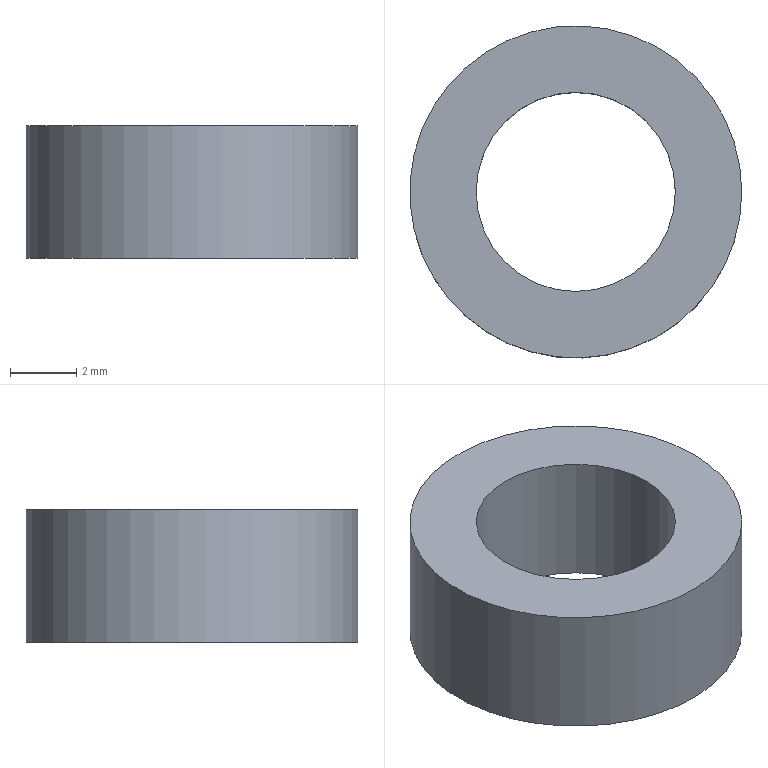Component | NX | BOTTOM_PLATE_WASHER | 1 solid | 4 faces | box 10 x 10 x 4 mm | volume 201 mm3 | cylinder 2 | plane 2 | commonest cylinder face diameters 10 x1 6 x1
STEP:
#1=CARTESIAN_POINT('',(0.,0.,0.));
#2=DIRECTION('',(0.,0.,1.));
#3=DIRECTION('',(1.,0.,0.));
#4=AXIS2_PLACEMENT_3D('',#1,#2,#3);
#5=CARTESIAN_POINT('',(5.,-10.,117.5));
#6=VERTEX_POINT('',#5);
#7=CARTESIAN_POINT('',(-0.,-10.,117.5));
#8=DIRECTION('',(0.,0.,1.));
#9=DIRECTION('',(1.,0.,0.));
#10=AXIS2_PLACEMENT_3D('',#7,#8,#9);
#11=CIRCLE('',#10,5.);
#12=CARTESIAN_POINT('',(-0.,-10.,117.5));
#13=DIRECTION('',(0.,0.,1.));
#14=DIRECTION('',(-1.,0.,0.));
#15=AXIS2_PLACEMENT_3D('',#12,#13,#14);
#16=CYLINDRICAL_SURFACE('',#15,5.);
#17=CARTESIAN_POINT('',(3.142,0.));
#18=DIRECTION('',(1.,0.));
#19=VECTOR('',#18,1.);
#20=LINE('',#17,#19);
#21=(GEOMETRIC_REPRESENTATION_CONTEXT(2)PARAMETRIC_REPRESENTATION_CONTEXT()REPRESENTATION_CONTEXT('',''));
#22=DEFINITIONAL_REPRESENTATION('',(#20),#21);
#23=PCURVE('',#16,#22);
#24=CARTESIAN_POINT('',(-0.,-10.,117.5));
#25=DIRECTION('',(0.,0.,1.));
#26=DIRECTION('',(-1.,0.,0.));
#27=AXIS2_PLACEMENT_3D('',#24,#25,#26);
#28=PLANE('',#27);
#29=CARTESIAN_POINT('',(0.,0.));
#30=DIRECTION('',(-1.,0.));
#31=AXIS2_PLACEMENT_2D('',#29,#30);
#32=CIRCLE('',#31,5.);
#33=(GEOMETRIC_REPRESENTATION_CONTEXT(2)PARAMETRIC_REPRESENTATION_CONTEXT()REPRESENTATION_CONTEXT('',''));
#34=DEFINITIONAL_REPRESENTATION('',(#32),#33);
#35=PCURVE('',#28,#34);
#36=SURFACE_CURVE('',#11,(#23,#35),.PCURVE_S1.);
#37=EDGE_CURVE('',#6,#6,#36,.T.);
#38=ORIENTED_EDGE('',*,*,#37,.T.);
#39=CARTESIAN_POINT('',(5.,-10.,121.5));
#40=VERTEX_POINT('',#39);
#41=CARTESIAN_POINT('',(5.,-10.,117.5));
#42=CARTESIAN_POINT('',(5.,-10.,121.5));
#43=B_SPLINE_CURVE_WITH_KNOTS('',1,(#41,#42),.UNSPECIFIED.,.F.,.F.,(2,2),(0.,4.),.PIECEWISE_BEZIER_KNOTS.);
#44=CARTESIAN_POINT('',(9.425,0.));
#45=DIRECTION('',(0.,1.));
#46=VECTOR('',#45,1.);
#47=LINE('',#44,#46);
#48=(GEOMETRIC_REPRESENTATION_CONTEXT(2)PARAMETRIC_REPRESENTATION_CONTEXT()REPRESENTATION_CONTEXT('',''));
#49=DEFINITIONAL_REPRESENTATION('',(#47),#48);
#50=PCURVE('',#16,#49);
#51=CARTESIAN_POINT('',(3.142,0.));
#52=DIRECTION('',(0.,1.));
#53=VECTOR('',#52,1.);
#54=LINE('',#51,#53);
#55=(GEOMETRIC_REPRESENTATION_CONTEXT(2)PARAMETRIC_REPRESENTATION_CONTEXT()REPRESENTATION_CONTEXT('',''));
#56=DEFINITIONAL_REPRESENTATION('',(#54),#55);
#57=PCURVE('',#16,#56);
#58=SEAM_CURVE('',#43,(#50,#57),.PCURVE_S1.);
#59=EDGE_CURVE('',#6,#40,#58,.T.);
#60=ORIENTED_EDGE('',*,*,#59,.T.);
#61=CARTESIAN_POINT('',(-0.,-10.,121.5));
#62=DIRECTION('',(0.,0.,1.));
#63=DIRECTION('',(1.,0.,0.));
#64=AXIS2_PLACEMENT_3D('',#61,#62,#63);
#65=CIRCLE('',#64,5.);
#66=CARTESIAN_POINT('',(3.142,4.));
#67=DIRECTION('',(1.,0.));
#68=VECTOR('',#67,1.);
#69=LINE('',#66,#68);
#70=(GEOMETRIC_REPRESENTATION_CONTEXT(2)PARAMETRIC_REPRESENTATION_CONTEXT()REPRESENTATION_CONTEXT('',''));
#71=DEFINITIONAL_REPRESENTATION('',(#69),#70);
#72=PCURVE('',#16,#71);
#73=CARTESIAN_POINT('',(-0.,-10.,121.5));
#74=DIRECTION('',(0.,0.,1.));
#75=DIRECTION('',(-1.,0.,0.));
#76=AXIS2_PLACEMENT_3D('',#73,#74,#75);
#77=PLANE('',#76);
#78=CARTESIAN_POINT('',(0.,0.));
#79=DIRECTION('',(-1.,0.));
#80=AXIS2_PLACEMENT_2D('',#78,#79);
#81=CIRCLE('',#80,5.);
#82=(GEOMETRIC_REPRESENTATION_CONTEXT(2)PARAMETRIC_REPRESENTATION_CONTEXT()REPRESENTATION_CONTEXT('',''));
#83=DEFINITIONAL_REPRESENTATION('',(#81),#82);
#84=PCURVE('',#77,#83);
#85=SURFACE_CURVE('',#65,(#72,#84),.PCURVE_S1.);
#86=EDGE_CURVE('',#40,#40,#85,.T.);
#87=ORIENTED_EDGE('',*,*,#86,.F.);
#88=ORIENTED_EDGE('',*,*,#59,.F.);
#89=EDGE_LOOP('',(#38,#60,#87,#88));
#90=FACE_BOUND('',#89,.T.);
#91=ADVANCED_FACE('',(#90),#16,.T.);
#92=CARTESIAN_POINT('',(3.,-10.,117.5));
#93=VERTEX_POINT('',#92);
#94=CARTESIAN_POINT('',(-0.,-10.,117.5));
#95=DIRECTION('',(0.,0.,1.));
#96=DIRECTION('',(1.,0.,0.));
#97=AXIS2_PLACEMENT_3D('',#94,#95,#96);
#98=CIRCLE('',#97,3.);
#99=CARTESIAN_POINT('',(-0.,-10.,117.5));
#100=DIRECTION('',(0.,0.,1.));
#101=DIRECTION('',(-1.,0.,0.));
#102=AXIS2_PLACEMENT_3D('',#99,#100,#101);
#103=CYLINDRICAL_SURFACE('',#102,3.);
#104=CARTESIAN_POINT('',(3.142,0.));
#105=DIRECTION('',(1.,0.));
#106=VECTOR('',#105,1.);
#107=LINE('',#104,#106);
#108=(GEOMETRIC_REPRESENTATION_CONTEXT(2)PARAMETRIC_REPRESENTATION_CONTEXT()REPRESENTATION_CONTEXT('',''));
#109=DEFINITIONAL_REPRESENTATION('',(#107),#108);
#110=PCURVE('',#103,#109);
#111=CARTESIAN_POINT('',(0.,0.));
#112=DIRECTION('',(-1.,0.));
#113=AXIS2_PLACEMENT_2D('',#111,#112);
#114=CIRCLE('',#113,3.);
#115=(GEOMETRIC_REPRESENTATION_CONTEXT(2)PARAMETRIC_REPRESENTATION_CONTEXT()REPRESENTATION_CONTEXT('',''));
#116=DEFINITIONAL_REPRESENTATION('',(#114),#115);
#117=PCURVE('',#28,#116);
#118=SURFACE_CURVE('',#98,(#110,#117),.PCURVE_S1.);
#119=EDGE_CURVE('',#93,#93,#118,.T.);
#120=ORIENTED_EDGE('',*,*,#119,.T.);
#121=CARTESIAN_POINT('',(3.,-10.,121.5));
#122=VERTEX_POINT('',#121);
#123=CARTESIAN_POINT('',(3.,-10.,117.5));
#124=CARTESIAN_POINT('',(3.,-10.,121.5));
#125=B_SPLINE_CURVE_WITH_KNOTS('',1,(#123,#124),.UNSPECIFIED.,.F.,.F.,(2,2),(0.,4.),.PIECEWISE_BEZIER_KNOTS.);
#126=CARTESIAN_POINT('',(9.425,0.));
#127=DIRECTION('',(0.,1.));
#128=VECTOR('',#127,1.);
#129=LINE('',#126,#128);
#130=(GEOMETRIC_REPRESENTATION_CONTEXT(2)PARAMETRIC_REPRESENTATION_CONTEXT()REPRESENTATION_CONTEXT('',''));
#131=DEFINITIONAL_REPRESENTATION('',(#129),#130);
#132=PCURVE('',#103,#131);
#133=CARTESIAN_POINT('',(3.142,0.));
#134=DIRECTION('',(0.,1.));
#135=VECTOR('',#134,1.);
#136=LINE('',#133,#135);
#137=(GEOMETRIC_REPRESENTATION_CONTEXT(2)PARAMETRIC_REPRESENTATION_CONTEXT()REPRESENTATION_CONTEXT('',''));
#138=DEFINITIONAL_REPRESENTATION('',(#136),#137);
#139=PCURVE('',#103,#138);
#140=SEAM_CURVE('',#125,(#132,#139),.PCURVE_S1.);
#141=EDGE_CURVE('',#93,#122,#140,.T.);
#142=ORIENTED_EDGE('',*,*,#141,.T.);
#143=CARTESIAN_POINT('',(-0.,-10.,121.5));
#144=DIRECTION('',(0.,0.,1.));
#145=DIRECTION('',(1.,0.,0.));
#146=AXIS2_PLACEMENT_3D('',#143,#144,#145);
#147=CIRCLE('',#146,3.);
#148=CARTESIAN_POINT('',(3.142,4.));
#149=DIRECTION('',(1.,0.));
#150=VECTOR('',#149,1.);
#151=LINE('',#148,#150);
#152=(GEOMETRIC_REPRESENTATION_CONTEXT(2)PARAMETRIC_REPRESENTATION_CONTEXT()REPRESENTATION_CONTEXT('',''));
#153=DEFINITIONAL_REPRESENTATION('',(#151),#152);
#154=PCURVE('',#103,#153);
#155=CARTESIAN_POINT('',(0.,0.));
#156=DIRECTION('',(-1.,0.));
#157=AXIS2_PLACEMENT_2D('',#155,#156);
#158=CIRCLE('',#157,3.);
#159=(GEOMETRIC_REPRESENTATION_CONTEXT(2)PARAMETRIC_REPRESENTATION_CONTEXT()REPRESENTATION_CONTEXT('',''));
#160=DEFINITIONAL_REPRESENTATION('',(#158),#159);
#161=PCURVE('',#77,#160);
#162=SURFACE_CURVE('',#147,(#154,#161),.PCURVE_S1.);
#163=EDGE_CURVE('',#122,#122,#162,.T.);
#164=ORIENTED_EDGE('',*,*,#163,.F.);
#165=ORIENTED_EDGE('',*,*,#141,.F.);
#166=EDGE_LOOP('',(#120,#142,#164,#165));
#167=FACE_BOUND('',#166,.F.);
#168=ADVANCED_FACE('',(#167),#103,.F.);
#169=ORIENTED_EDGE('',*,*,#37,.F.);
#170=EDGE_LOOP('',(#169));
#171=FACE_BOUND('',#170,.T.);
#172=ORIENTED_EDGE('',*,*,#119,.T.);
#173=EDGE_LOOP('',(#172));
#174=FACE_BOUND('',#173,.T.);
#175=ADVANCED_FACE('',(#171,#174),#28,.F.);
#176=ORIENTED_EDGE('',*,*,#86,.T.);
#177=EDGE_LOOP('',(#176));
#178=FACE_BOUND('',#177,.T.);
#179=ORIENTED_EDGE('',*,*,#163,.F.);
#180=EDGE_LOOP('',(#179));
#181=FACE_BOUND('',#180,.T.);
#182=ADVANCED_FACE('',(#178,#181),#77,.T.);
#183=CLOSED_SHELL('',(#91,#168,#175,#182));
#184=MANIFOLD_SOLID_BREP('',#183);
#185=(LENGTH_UNIT()NAMED_UNIT(*)SI_UNIT(.MILLI.,.METRE.));
#186=UNCERTAINTY_MEASURE_WITH_UNIT(LENGTH_MEASURE(0.00001),#185,'','');
#187=(NAMED_UNIT(*)PLANE_ANGLE_UNIT()SI_UNIT($,.RADIAN.));
#188=(NAMED_UNIT(*)SI_UNIT($,.STERADIAN.)SOLID_ANGLE_UNIT());
#189=(GEOMETRIC_REPRESENTATION_CONTEXT(3)GLOBAL_UNCERTAINTY_ASSIGNED_CONTEXT((#186))GLOBAL_UNIT_ASSIGNED_CONTEXT((#185,#187,#188))REPRESENTATION_CONTEXT('',''));
#190=ADVANCED_BREP_SHAPE_REPRESENTATION('',(#4,#184),#189);